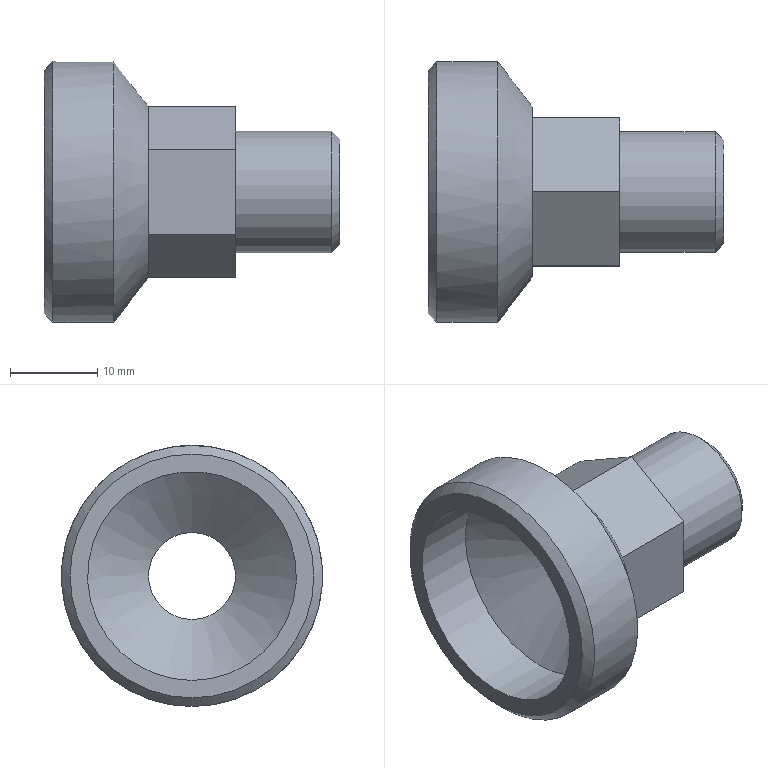Component | NX | 6_OIL_CUP_BODY | 1 solid | 29 faces | volume 5742 mm3 | plane 21 | cylinder 4 | cone 4 | commonest cylinder face diameters 10 x1 14 x1 30 x1 24 x1